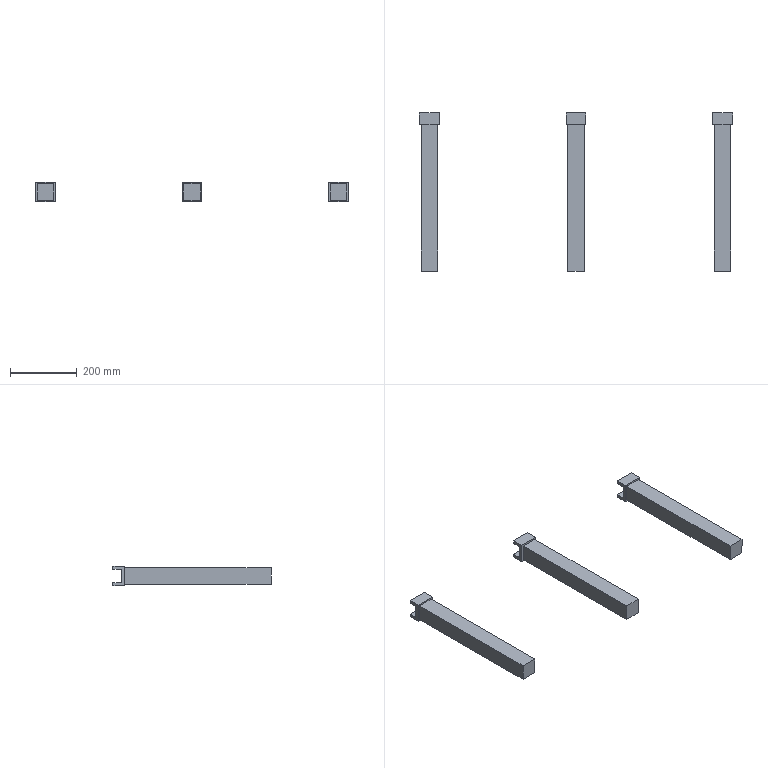Component | SolidWorks | OuterRodSupport-1 | 5 solids | 51 faces | box 940 x 475 x 60 mm | volume 3498003 mm3 | plane 51
build123d program:
from build123d import *

# Parameters (mm, degrees)
SKETCH1_W             = 50
SKETCH1_H             = 50
BOSS_EXTRUDE1_DEPTH   = 440
BOSS_EXTRUDE1_2_DEPTH = 440
BOSS_EXTRUDE1_3_DEPTH = 440
SKETCH2_W             = 60
SKETCH2_H             = 60
BOSS_EXTRUDE2_DEPTH   = 10
SKETCH3_W             = 60
SKETCH3_H             = 10
BOSS_EXTRUDE3_DEPTH   = 25


with BuildPart() as part:
    # Sketch1 → Boss-Extrude1 (new body)
    with BuildSketch(Plane.XY):
        with Locations((-440, 182.763)):
            Rectangle(SKETCH1_W, SKETCH1_H)
    extrude(amount=BOSS_EXTRUDE1_DEPTH)

    # Sketch2 → Boss-Extrude2 (add)
    with BuildSketch(Plane.XY.offset(440)):
        with Locations((-440, 182.763)):
            Rectangle(SKETCH2_W, SKETCH2_H)
        with Locations((0, 182.763)):
            Rectangle(SKETCH2_W, SKETCH2_H)
        with Locations((440, 182.763)):
            Rectangle(SKETCH2_W, SKETCH2_H)
    extrude(amount=BOSS_EXTRUDE2_DEPTH)


with BuildPart() as body_2:
    # Sketch1 → Boss-Extrude1 2 (new body)
    with BuildSketch(Plane.XY):
        with Locations((0, 182.763)):
            Rectangle(SKETCH1_W, SKETCH1_H)
    extrude(amount=BOSS_EXTRUDE1_2_DEPTH)


with BuildPart() as body_3:
    # Sketch1 → Boss-Extrude1 3 (new body)
    with BuildSketch(Plane.XY):
        with Locations((440, 182.763)):
            Rectangle(SKETCH1_W, SKETCH1_H)
    extrude(amount=BOSS_EXTRUDE1_3_DEPTH)


with BuildPart() as boss_extrude2_piece_1:
    # of the separate pieces the step leaves, piece 1, a body of its own (boss_extrude2_pieces)
    add(part.part.solids().sort_by_distance((-470, 152.763, 440))[0])



with BuildPart() as boss_extrude2_piece_2:
    # of the separate pieces the step leaves, piece 2, a body of its own (boss_extrude2_pieces)
    add(part.part.solids().sort_by_distance((-30, 152.763, 440))[0])


with BuildPart() as boss_extrude2_piece_3:
    # of the separate pieces the step leaves, piece 3, a body of its own (boss_extrude2_pieces)
    add(part.part.solids().sort_by_distance((410, 152.763, 440))[0])


with BuildPart() as boss_extrude2_piece_1_1:
    add(boss_extrude2_piece_1.part)

    add(boss_extrude2_piece_2.part)  # Boss-Extrude3 merges Boss-Extrude2 piece 2

    add(boss_extrude2_piece_3.part)  # Boss-Extrude3 merges Boss-Extrude2 piece 3
    # Sketch3 → Boss-Extrude3 (add)
    with BuildSketch(Plane.XY.offset(450)):
        with Locations((-440, 207.763)):
            Rectangle(SKETCH3_W, SKETCH3_H)
        with Locations((-440, 157.763)):
            Rectangle(SKETCH3_W, SKETCH3_H)
        with Locations((0, 157.763)):
            Rectangle(SKETCH3_W, SKETCH3_H)
        Polygon((-30, 212.763), (-30.01, 202.763), (30, 202.763), (30, 212.763), align=None)
        with Locations((440, 157.763)):
            Rectangle(SKETCH3_W, SKETCH3_H)
        Polygon((410, 212.763), (409.99, 202.763), (470, 202.763), (470, 212.763), align=None)
    extrude(amount=BOSS_EXTRUDE3_DEPTH)


solid = Compound([body_2.part, body_3.part, boss_extrude2_piece_1_1.part])

# Placed as in the assembly
solid = solid.moved(Location((0, 0, 0), (-90, 0, 0)))